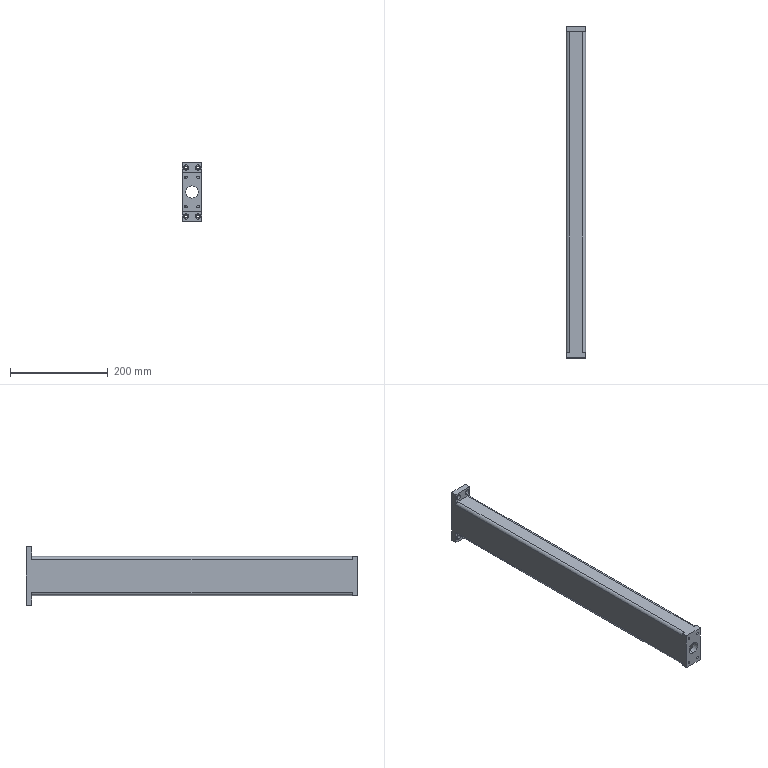Component | SolidWorks | A067-6 | 1 solid | 75 faces | box 40 x 679 x 120 mm | volume 646342 mm3 | cylinder 46 | plane 25 | cone 4 | commonest cylinder face diameters 5 x8 11 x8 6.4 x8 12 x6 4.2 x4 25 x4 4 x4 7 x2
build123d program:
from build123d import *

# Parameters (mm, degrees)
BOSS_EXTRUDE1_DEPTH                             = 655
SKETCH5_W                                       = 80
SKETCH5_H                                       = 65
BOSS_EXTRUDE4_DEPTH                             = 12
SKETCH6_W                                       = 120
SKETCH6_H                                       = 40
BOSS_EXTRUDE5_DEPTH                             = 12
M6_HEX_SOCKET_HEAD_CAP_SCREW_CBORE1_D           = 6.4
M6_HEX_SOCKET_HEAD_CAP_SCREW_CBORE1_CBORE_D     = 11
M6_HEX_SOCKET_HEAD_CAP_SCREW_CBORE1_CBORE_DEPTH = 6.4
F_5_0_5_DIAMETER_HOLE1_D                        = 5
F_5_0_5_DIAMETER_HOLE1_DEPTH                    = 10
F_5_0_5_DIAMETER_HOLE1_TIP                      = 1.502
M6_TAPPED_HOLE1_D                               = 5
M6_TAPPED_HOLE1_DEPTH                           = 17
M6_TAPPED_HOLE1_TIP                             = 1.502
SKETCH13_W                                      = 80
SKETCH13_H                                      = 12
CUT_EXTRUDE1_DEPTH                              = 25
SKETCH14_R                                      = 12.5
CUT_EXTRUDE2_DEPTH                              = 682.939
CUT_EXTRUDE3_REACH                              = 672.887
SKETCH15_R                                      = 6
M5_TAPPED_HOLE1_D                               = 4.2
M5_TAPPED_HOLE1_DEPTH                           = 4
SKETCH1_R                                       = 16
CYLINDER_END_RELIEF_DEPTH                       = 2.5
SKETCH2_R                                       = 3.5
LIMIT_BOLT_CLEARANCE_DEPTH                      = 5


with BuildPart() as part:
    # Sketch1_2 → Boss-Extrude1 (new body)
    with BuildSketch(Plane.XY):
        with BuildLine():
            Line((-34, 20), (34, 20))
            ThreePointArc((34, 20), (38.243, 18.243), (40, 14))
            Line((40, 14), (40, -14))
            ThreePointArc((40, -14), (38.243, -18.243), (34, -20))
            Line((34, -20), (-34, -20))
            ThreePointArc((-34, -20), (-38.243, -18.243), (-40, -14))
            Line((-40, -14), (-40, 14))
            ThreePointArc((-40, 14), (-38.243, 18.243), (-34, 20))
        make_face()
        with BuildLine():
            Line((-34, 16), (34, 16))
            ThreePointArc((34, 16), (35.414, 15.414), (36, 14))
            Line((36, 14), (36, -14))
            ThreePointArc((36, -14), (35.414, -15.414), (34, -16))
            Line((34, -16), (-34, -16))
            ThreePointArc((-34, -16), (-35.414, -15.414), (-36, -14))
            Line((-36, -14), (-36, 14))
            ThreePointArc((-36, 14), (-35.414, 15.414), (-34, 16))
        make_face(mode=Mode.SUBTRACT)
    extrude(amount=BOSS_EXTRUDE1_DEPTH)

    # Sketch5 → Boss-Extrude4 (add)
    with BuildSketch(Plane.XY.offset(655)):
        with Locations((0, 12.5)):
            Rectangle(SKETCH5_W, SKETCH5_H)
    extrude(amount=BOSS_EXTRUDE4_DEPTH)

    # Sketch6 → Boss-Extrude5 (add)
    with BuildSketch(Plane(origin=(0, 0, 0), x_dir=(-1, 0, 0), z_dir=(0, 0, -1))):
        Rectangle(SKETCH6_W, SKETCH6_H)
    extrude(amount=BOSS_EXTRUDE5_DEPTH)

    # M6 Hex Socket Head Cap Screw CBORE1 (through all)
    with Locations(Plane.XY):
        with Locations((50, -12.5), (50, 12.5), (-50, -12.5), (-50, 12.5)):
            CounterBoreHole(M6_HEX_SOCKET_HEAD_CAP_SCREW_CBORE1_D / 2, M6_HEX_SOCKET_HEAD_CAP_SCREW_CBORE1_CBORE_D / 2, M6_HEX_SOCKET_HEAD_CAP_SCREW_CBORE1_CBORE_DEPTH)

    # 5.0 _5_ Diameter Hole1
    with Locations(Plane.XY.offset(667)):
        with Locations((-30, 12.5), (30, 12.5)):
            Hole(F_5_0_5_DIAMETER_HOLE1_D / 2, depth=F_5_0_5_DIAMETER_HOLE1_DEPTH)
            with Locations((0, 0, -(F_5_0_5_DIAMETER_HOLE1_DEPTH + F_5_0_5_DIAMETER_HOLE1_TIP / 2))):  # 118° drill point
                Cone(0, F_5_0_5_DIAMETER_HOLE1_D / 2, F_5_0_5_DIAMETER_HOLE1_TIP, mode=Mode.SUBTRACT)

    # M6 Tapped Hole1
    with Locations(Plane.XY.offset(667)):
        with Locations((-30, 37.5), (30, 37.5), (-30, -12.5), (30, -12.5)):
            Hole(M6_TAPPED_HOLE1_D / 2, depth=M6_TAPPED_HOLE1_DEPTH)
            with Locations((0, 0, -(M6_TAPPED_HOLE1_DEPTH + M6_TAPPED_HOLE1_TIP / 2))):  # 118° drill point
                Cone(0, M6_TAPPED_HOLE1_D / 2, M6_TAPPED_HOLE1_TIP, mode=Mode.SUBTRACT)

    # Sketch13 → Cut-Extrude1 (cut)
    with BuildSketch(Plane(origin=(0, 45, 0), x_dir=(1, 0, 0), z_dir=(0, 1, 0))):
        with Locations((0, -661)):
            Rectangle(SKETCH13_W, SKETCH13_H)
    extrude(amount=-CUT_EXTRUDE1_DEPTH, mode=Mode.SUBTRACT)

    # Sketch14 → Cut-Extrude2 (cut, through all)
    with BuildSketch(Plane.XY.offset(667)):
        Circle(SKETCH14_R)
    extrude(amount=-CUT_EXTRUDE2_DEPTH, mode=Mode.SUBTRACT)

    # Sketch15 → Cut-Extrude3 (cut, up to next)
    with BuildSketch(Plane.XZ.offset(20), mode=Mode.PRIVATE) as cut_extrude3_sk1:
        with Locations((0, 620)):
            Circle(SKETCH15_R)
    cut_extrude3_tool1 = extrude(cut_extrude3_sk1.sketch, amount=-CUT_EXTRUDE3_REACH, mode=Mode.PRIVATE) & part.part
    add(cut_extrude3_tool1.solids().sort_by_distance((0, -20, 620))[0], mode=Mode.SUBTRACT)

    # M5 Tapped Hole1
    with Locations(Plane(origin=(0, -20, 0), x_dir=(-1, 0, 0), z_dir=(0, -1, 0))):
        with Locations((25, -606), (-25, -606)):
            Hole(M5_TAPPED_HOLE1_D / 2, depth=M5_TAPPED_HOLE1_DEPTH)

    # Sketch1 → Cylinder End Relief (cut)
    with BuildSketch(Plane.XZ.offset(20)):
        with Locations((-18.5, 646)):
            Circle(SKETCH1_R)
    extrude(amount=-CYLINDER_END_RELIEF_DEPTH, mode=Mode.SUBTRACT)

    # Sketch2 → Limit Bolt Clearance (cut)
    with BuildSketch(Plane.XZ.offset(20)):
        with Locations((15, 643.5)):
            Circle(SKETCH2_R)
    extrude(amount=-LIMIT_BOLT_CLEARANCE_DEPTH, mode=Mode.SUBTRACT)


solid = part.part

# Placed as in the assembly
solid = solid.moved(Location((696.381, 667, 60), (90, 0, 90)))